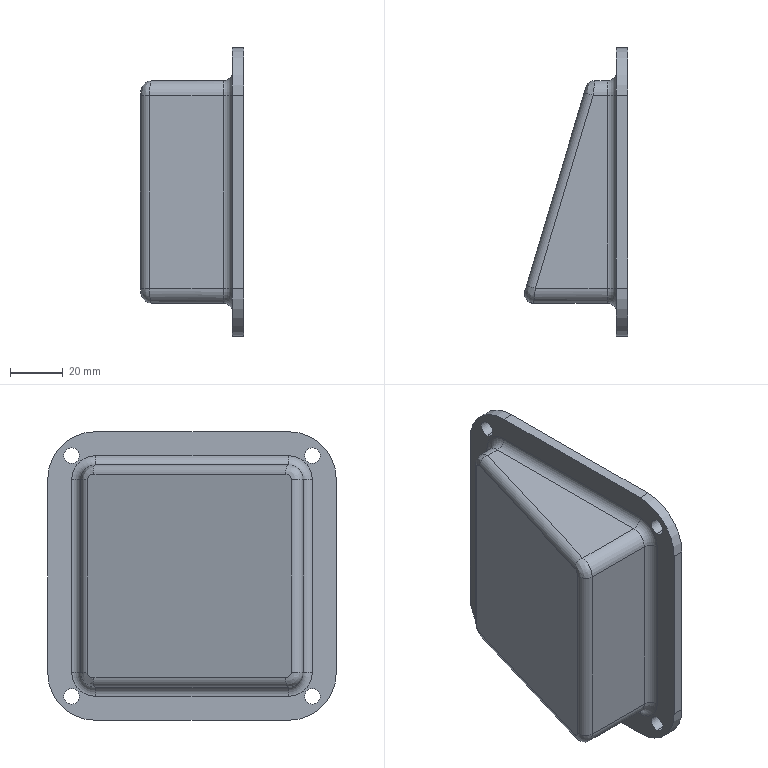Component | SolidWorks | Three-PhaseAsynchronousMotor-1_MotorJunctionBox-1 | 1 solid | 52 faces | volume 189044 mm3 | cylinder 28 | plane 16 | spline 4 | torus 4 | commonest cylinder face diameters 5.95 x8 7 x8 11.2 x4 36.4 x4 5.6 x4